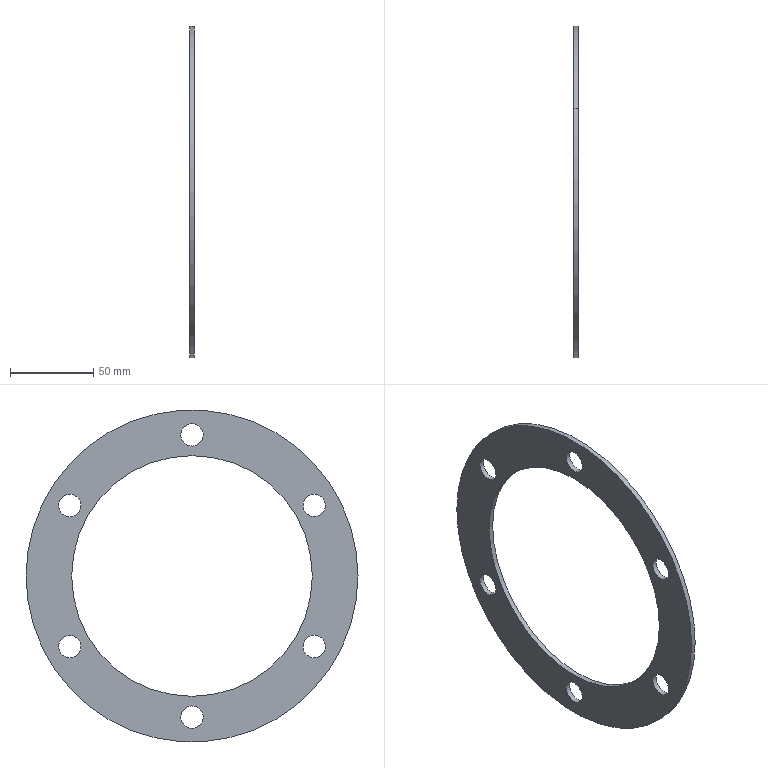Component | SolidWorks | JF21-80.1-33-1-SOLID1-1 | 1 solid | 18 faces | box 3 x 200 x 200 mm | volume 42132 mm3 | cylinder 16 | plane 2 | commonest cylinder face diameters 13.5 x12 145 x2 200 x2
STEP:
#1=COLOUR_RGB('',0.7922,0.8196,0.9333);
#2=FILL_AREA_STYLE_COLOUR('',#1);
#3=FILL_AREA_STYLE('',(#2));
#4=SURFACE_STYLE_FILL_AREA(#3);
#5=SURFACE_SIDE_STYLE('',(#4));
#6=SURFACE_STYLE_USAGE(.BOTH.,#5);
#7=PRESENTATION_STYLE_ASSIGNMENT((#6));
#8=CARTESIAN_POINT('',(17.244,-0.1329,18.038));
#9=VERTEX_POINT('',#8);
#10=CARTESIAN_POINT('',(17.244,0.1329,18.498));
#11=VERTEX_POINT('',#10);
#12=CARTESIAN_POINT('',(17.244,0.,18.268));
#13=DIRECTION('',(-1.,0.,0.));
#14=DIRECTION('',(0.,0.5,0.866));
#15=AXIS2_PLACEMENT_3D('',#12,#13,#14);
#16=CIRCLE('',#15,0.2657);
#17=EDGE_CURVE('',#9,#11,#16,.T.);
#18=ORIENTED_EDGE('',*,*,#17,.F.);
#19=CARTESIAN_POINT('',(17.126,-0.1329,18.038));
#20=VERTEX_POINT('',#19);
#21=CARTESIAN_POINT('',(17.126,-0.1329,18.038));
#22=DIRECTION('',(-1.,0.,0.));
#23=VECTOR('',#22,39.37);
#24=LINE('',#21,#23);
#25=EDGE_CURVE('',#9,#20,#24,.T.);
#26=ORIENTED_EDGE('',*,*,#25,.T.);
#27=CARTESIAN_POINT('',(17.126,0.1329,18.498));
#28=VERTEX_POINT('',#27);
#29=CARTESIAN_POINT('',(17.126,0.,18.268));
#30=DIRECTION('',(-1.,0.,0.));
#31=DIRECTION('',(0.,0.5,0.866));
#32=AXIS2_PLACEMENT_3D('',#29,#30,#31);
#33=CIRCLE('',#32,0.2657);
#34=EDGE_CURVE('',#20,#28,#33,.T.);
#35=ORIENTED_EDGE('',*,*,#34,.T.);
#36=CARTESIAN_POINT('',(17.126,0.1329,18.498));
#37=DIRECTION('',(-1.,0.,0.));
#38=VECTOR('',#37,39.37);
#39=LINE('',#36,#38);
#40=EDGE_CURVE('',#11,#28,#39,.T.);
#41=ORIENTED_EDGE('',*,*,#40,.F.);
#42=EDGE_LOOP('',(#18,#26,#35,#41));
#43=FACE_OUTER_BOUND('',#42,.T.);
#44=CARTESIAN_POINT('',(17.126,0.,18.268));
#45=DIRECTION('',(-1.,0.,0.));
#46=DIRECTION('',(0.,-0.5,-0.866));
#47=AXIS2_PLACEMENT_3D('',#44,#45,#46);
#48=CYLINDRICAL_SURFACE('',#47,0.2657);
#49=ADVANCED_FACE('',(#43),#48,.F.);
#50=CARTESIAN_POINT('',(17.244,-3.031,19.711));
#51=VERTEX_POINT('',#50);
#52=CARTESIAN_POINT('',(17.244,-2.765,20.171));
#53=VERTEX_POINT('',#52);
#54=CARTESIAN_POINT('',(17.244,-2.898,19.941));
#55=DIRECTION('',(-1.,0.,0.));
#56=DIRECTION('',(0.,0.5,0.866));
#57=AXIS2_PLACEMENT_3D('',#54,#55,#56);
#58=CIRCLE('',#57,0.2657);
#59=EDGE_CURVE('',#51,#53,#58,.T.);
#60=ORIENTED_EDGE('',*,*,#59,.F.);
#61=CARTESIAN_POINT('',(17.126,-3.031,19.711));
#62=VERTEX_POINT('',#61);
#63=CARTESIAN_POINT('',(17.126,-3.031,19.711));
#64=DIRECTION('',(-1.,0.,0.));
#65=VECTOR('',#64,39.37);
#66=LINE('',#63,#65);
#67=EDGE_CURVE('',#51,#62,#66,.T.);
#68=ORIENTED_EDGE('',*,*,#67,.T.);
#69=CARTESIAN_POINT('',(17.126,-2.765,20.171));
#70=VERTEX_POINT('',#69);
#71=CARTESIAN_POINT('',(17.126,-2.898,19.941));
#72=DIRECTION('',(-1.,0.,0.));
#73=DIRECTION('',(0.,0.5,0.866));
#74=AXIS2_PLACEMENT_3D('',#71,#72,#73);
#75=CIRCLE('',#74,0.2657);
#76=EDGE_CURVE('',#62,#70,#75,.T.);
#77=ORIENTED_EDGE('',*,*,#76,.T.);
#78=CARTESIAN_POINT('',(17.126,-2.765,20.171));
#79=DIRECTION('',(-1.,0.,0.));
#80=VECTOR('',#79,39.37);
#81=LINE('',#78,#80);
#82=EDGE_CURVE('',#53,#70,#81,.T.);
#83=ORIENTED_EDGE('',*,*,#82,.F.);
#84=EDGE_LOOP('',(#60,#68,#77,#83));
#85=FACE_OUTER_BOUND('',#84,.T.);
#86=CARTESIAN_POINT('',(17.126,-2.898,19.941));
#87=DIRECTION('',(-1.,0.,0.));
#88=DIRECTION('',(0.,-0.5,-0.866));
#89=AXIS2_PLACEMENT_3D('',#86,#87,#88);
#90=CYLINDRICAL_SURFACE('',#89,0.2657);
#91=ADVANCED_FACE('',(#85),#90,.F.);
#92=CARTESIAN_POINT('',(17.244,-3.031,23.057));
#93=VERTEX_POINT('',#92);
#94=CARTESIAN_POINT('',(17.244,-2.765,23.518));
#95=VERTEX_POINT('',#94);
#96=CARTESIAN_POINT('',(17.244,-2.898,23.287));
#97=DIRECTION('',(-1.,0.,0.));
#98=DIRECTION('',(0.,0.5,0.866));
#99=AXIS2_PLACEMENT_3D('',#96,#97,#98);
#100=CIRCLE('',#99,0.2657);
#101=EDGE_CURVE('',#93,#95,#100,.T.);
#102=ORIENTED_EDGE('',*,*,#101,.F.);
#103=CARTESIAN_POINT('',(17.126,-3.031,23.057));
#104=VERTEX_POINT('',#103);
#105=CARTESIAN_POINT('',(17.126,-3.031,23.057));
#106=DIRECTION('',(-1.,0.,0.));
#107=VECTOR('',#106,39.37);
#108=LINE('',#105,#107);
#109=EDGE_CURVE('',#93,#104,#108,.T.);
#110=ORIENTED_EDGE('',*,*,#109,.T.);
#111=CARTESIAN_POINT('',(17.126,-2.765,23.518));
#112=VERTEX_POINT('',#111);
#113=CARTESIAN_POINT('',(17.126,-2.898,23.287));
#114=DIRECTION('',(-1.,0.,0.));
#115=DIRECTION('',(0.,0.5,0.866));
#116=AXIS2_PLACEMENT_3D('',#113,#114,#115);
#117=CIRCLE('',#116,0.2657);
#118=EDGE_CURVE('',#104,#112,#117,.T.);
#119=ORIENTED_EDGE('',*,*,#118,.T.);
#120=CARTESIAN_POINT('',(17.126,-2.765,23.518));
#121=DIRECTION('',(-1.,0.,0.));
#122=VECTOR('',#121,39.37);
#123=LINE('',#120,#122);
#124=EDGE_CURVE('',#95,#112,#123,.T.);
#125=ORIENTED_EDGE('',*,*,#124,.F.);
#126=EDGE_LOOP('',(#102,#110,#119,#125));
#127=FACE_OUTER_BOUND('',#126,.T.);
#128=CARTESIAN_POINT('',(17.126,-2.898,23.287));
#129=DIRECTION('',(-1.,0.,0.));
#130=DIRECTION('',(0.,-0.5,-0.866));
#131=AXIS2_PLACEMENT_3D('',#128,#129,#130);
#132=CYLINDRICAL_SURFACE('',#131,0.2657);
#133=ADVANCED_FACE('',(#127),#132,.F.);
#134=CARTESIAN_POINT('',(17.244,-0.1329,24.73));
#135=VERTEX_POINT('',#134);
#136=CARTESIAN_POINT('',(17.244,0.1329,25.191));
#137=VERTEX_POINT('',#136);
#138=CARTESIAN_POINT('',(17.244,0.,24.961));
#139=DIRECTION('',(-1.,0.,0.));
#140=DIRECTION('',(0.,0.5,0.866));
#141=AXIS2_PLACEMENT_3D('',#138,#139,#140);
#142=CIRCLE('',#141,0.2657);
#143=EDGE_CURVE('',#135,#137,#142,.T.);
#144=ORIENTED_EDGE('',*,*,#143,.F.);
#145=CARTESIAN_POINT('',(17.126,-0.1329,24.73));
#146=VERTEX_POINT('',#145);
#147=CARTESIAN_POINT('',(17.126,-0.1329,24.73));
#148=DIRECTION('',(-1.,0.,0.));
#149=VECTOR('',#148,39.37);
#150=LINE('',#147,#149);
#151=EDGE_CURVE('',#135,#146,#150,.T.);
#152=ORIENTED_EDGE('',*,*,#151,.T.);
#153=CARTESIAN_POINT('',(17.126,0.1329,25.191));
#154=VERTEX_POINT('',#153);
#155=CARTESIAN_POINT('',(17.126,0.,24.961));
#156=DIRECTION('',(-1.,0.,0.));
#157=DIRECTION('',(0.,0.5,0.866));
#158=AXIS2_PLACEMENT_3D('',#155,#156,#157);
#159=CIRCLE('',#158,0.2657);
#160=EDGE_CURVE('',#146,#154,#159,.T.);
#161=ORIENTED_EDGE('',*,*,#160,.T.);
#162=CARTESIAN_POINT('',(17.126,0.1329,25.191));
#163=DIRECTION('',(-1.,0.,0.));
#164=VECTOR('',#163,39.37);
#165=LINE('',#162,#164);
#166=EDGE_CURVE('',#137,#154,#165,.T.);
#167=ORIENTED_EDGE('',*,*,#166,.F.);
#168=EDGE_LOOP('',(#144,#152,#161,#167));
#169=FACE_OUTER_BOUND('',#168,.T.);
#170=CARTESIAN_POINT('',(17.126,0.,24.961));
#171=DIRECTION('',(-1.,0.,0.));
#172=DIRECTION('',(0.,-0.5,-0.866));
#173=AXIS2_PLACEMENT_3D('',#170,#171,#172);
#174=CYLINDRICAL_SURFACE('',#173,0.2657);
#175=ADVANCED_FACE('',(#169),#174,.F.);
#176=CARTESIAN_POINT('',(17.244,2.765,23.057));
#177=VERTEX_POINT('',#176);
#178=CARTESIAN_POINT('',(17.244,3.031,23.518));
#179=VERTEX_POINT('',#178);
#180=CARTESIAN_POINT('',(17.244,2.898,23.287));
#181=DIRECTION('',(-1.,0.,0.));
#182=DIRECTION('',(0.,0.5,0.866));
#183=AXIS2_PLACEMENT_3D('',#180,#181,#182);
#184=CIRCLE('',#183,0.2657);
#185=EDGE_CURVE('',#177,#179,#184,.T.);
#186=ORIENTED_EDGE('',*,*,#185,.F.);
#187=CARTESIAN_POINT('',(17.126,2.765,23.057));
#188=VERTEX_POINT('',#187);
#189=CARTESIAN_POINT('',(17.126,2.765,23.057));
#190=DIRECTION('',(-1.,0.,0.));
#191=VECTOR('',#190,39.37);
#192=LINE('',#189,#191);
#193=EDGE_CURVE('',#177,#188,#192,.T.);
#194=ORIENTED_EDGE('',*,*,#193,.T.);
#195=CARTESIAN_POINT('',(17.126,3.031,23.518));
#196=VERTEX_POINT('',#195);
#197=CARTESIAN_POINT('',(17.126,2.898,23.287));
#198=DIRECTION('',(-1.,0.,0.));
#199=DIRECTION('',(0.,0.5,0.866));
#200=AXIS2_PLACEMENT_3D('',#197,#198,#199);
#201=CIRCLE('',#200,0.2657);
#202=EDGE_CURVE('',#188,#196,#201,.T.);
#203=ORIENTED_EDGE('',*,*,#202,.T.);
#204=CARTESIAN_POINT('',(17.126,3.031,23.518));
#205=DIRECTION('',(-1.,0.,0.));
#206=VECTOR('',#205,39.37);
#207=LINE('',#204,#206);
#208=EDGE_CURVE('',#179,#196,#207,.T.);
#209=ORIENTED_EDGE('',*,*,#208,.F.);
#210=EDGE_LOOP('',(#186,#194,#203,#209));
#211=FACE_OUTER_BOUND('',#210,.T.);
#212=CARTESIAN_POINT('',(17.126,2.898,23.287));
#213=DIRECTION('',(-1.,0.,0.));
#214=DIRECTION('',(0.,-0.5,-0.866));
#215=AXIS2_PLACEMENT_3D('',#212,#213,#214);
#216=CYLINDRICAL_SURFACE('',#215,0.2657);
#217=ADVANCED_FACE('',(#211),#216,.F.);
#218=CARTESIAN_POINT('',(17.244,2.765,19.711));
#219=VERTEX_POINT('',#218);
#220=CARTESIAN_POINT('',(17.244,3.031,20.171));
#221=VERTEX_POINT('',#220);
#222=CARTESIAN_POINT('',(17.244,2.898,19.941));
#223=DIRECTION('',(-1.,0.,0.));
#224=DIRECTION('',(0.,0.5,0.866));
#225=AXIS2_PLACEMENT_3D('',#222,#223,#224);
#226=CIRCLE('',#225,0.2657);
#227=EDGE_CURVE('',#219,#221,#226,.T.);
#228=ORIENTED_EDGE('',*,*,#227,.F.);
#229=CARTESIAN_POINT('',(17.126,2.765,19.711));
#230=VERTEX_POINT('',#229);
#231=CARTESIAN_POINT('',(17.126,2.765,19.711));
#232=DIRECTION('',(-1.,0.,0.));
#233=VECTOR('',#232,39.37);
#234=LINE('',#231,#233);
#235=EDGE_CURVE('',#219,#230,#234,.T.);
#236=ORIENTED_EDGE('',*,*,#235,.T.);
#237=CARTESIAN_POINT('',(17.126,3.031,20.171));
#238=VERTEX_POINT('',#237);
#239=CARTESIAN_POINT('',(17.126,2.898,19.941));
#240=DIRECTION('',(-1.,0.,0.));
#241=DIRECTION('',(0.,0.5,0.866));
#242=AXIS2_PLACEMENT_3D('',#239,#240,#241);
#243=CIRCLE('',#242,0.2657);
#244=EDGE_CURVE('',#230,#238,#243,.T.);
#245=ORIENTED_EDGE('',*,*,#244,.T.);
#246=CARTESIAN_POINT('',(17.126,3.031,20.171));
#247=DIRECTION('',(-1.,0.,0.));
#248=VECTOR('',#247,39.37);
#249=LINE('',#246,#248);
#250=EDGE_CURVE('',#221,#238,#249,.T.);
#251=ORIENTED_EDGE('',*,*,#250,.F.);
#252=EDGE_LOOP('',(#228,#236,#245,#251));
#253=FACE_OUTER_BOUND('',#252,.T.);
#254=CARTESIAN_POINT('',(17.126,2.898,19.941));
#255=DIRECTION('',(-1.,0.,0.));
#256=DIRECTION('',(0.,-0.5,-0.866));
#257=AXIS2_PLACEMENT_3D('',#254,#255,#256);
#258=CYLINDRICAL_SURFACE('',#257,0.2657);
#259=ADVANCED_FACE('',(#253),#258,.F.);
#260=CARTESIAN_POINT('',(17.126,-1.427,19.142));
#261=VERTEX_POINT('',#260);
#262=CARTESIAN_POINT('',(17.126,1.427,24.086));
#263=VERTEX_POINT('',#262);
#264=CARTESIAN_POINT('',(17.126,0.,21.614));
#265=DIRECTION('',(-1.,0.,0.));
#266=DIRECTION('',(0.,0.5,0.866));
#267=AXIS2_PLACEMENT_3D('',#264,#265,#266);
#268=CIRCLE('',#267,2.854);
#269=EDGE_CURVE('',#261,#263,#268,.T.);
#270=ORIENTED_EDGE('',*,*,#269,.T.);
#271=CARTESIAN_POINT('',(17.244,1.427,24.086));
#272=VERTEX_POINT('',#271);
#273=CARTESIAN_POINT('',(17.126,1.427,24.086));
#274=DIRECTION('',(-1.,0.,0.));
#275=VECTOR('',#274,39.37);
#276=LINE('',#273,#275);
#277=EDGE_CURVE('',#272,#263,#276,.T.);
#278=ORIENTED_EDGE('',*,*,#277,.F.);
#279=CARTESIAN_POINT('',(17.244,-1.427,19.142));
#280=VERTEX_POINT('',#279);
#281=CARTESIAN_POINT('',(17.244,0.,21.614));
#282=DIRECTION('',(-1.,0.,0.));
#283=DIRECTION('',(0.,0.5,0.866));
#284=AXIS2_PLACEMENT_3D('',#281,#282,#283);
#285=CIRCLE('',#284,2.854);
#286=EDGE_CURVE('',#280,#272,#285,.T.);
#287=ORIENTED_EDGE('',*,*,#286,.F.);
#288=CARTESIAN_POINT('',(17.126,-1.427,19.142));
#289=DIRECTION('',(-1.,0.,0.));
#290=VECTOR('',#289,39.37);
#291=LINE('',#288,#290);
#292=EDGE_CURVE('',#280,#261,#291,.T.);
#293=ORIENTED_EDGE('',*,*,#292,.T.);
#294=EDGE_LOOP('',(#270,#278,#287,#293));
#295=FACE_OUTER_BOUND('',#294,.T.);
#296=CARTESIAN_POINT('',(17.126,0.,21.614));
#297=DIRECTION('',(1.,0.,0.));
#298=DIRECTION('',(0.,0.5,0.866));
#299=AXIS2_PLACEMENT_3D('',#296,#297,#298);
#300=CYLINDRICAL_SURFACE('',#299,2.854);
#301=ADVANCED_FACE('',(#295),#300,.F.);
#302=CARTESIAN_POINT('',(17.126,1.969,25.024));
#303=VERTEX_POINT('',#302);
#304=CARTESIAN_POINT('',(17.126,-1.969,18.205));
#305=VERTEX_POINT('',#304);
#306=CARTESIAN_POINT('',(17.126,0.,21.614));
#307=DIRECTION('',(-1.,0.,0.));
#308=DIRECTION('',(0.,0.5,0.866));
#309=AXIS2_PLACEMENT_3D('',#306,#307,#308);
#310=CIRCLE('',#309,3.937);
#311=EDGE_CURVE('',#303,#305,#310,.T.);
#312=ORIENTED_EDGE('',*,*,#311,.F.);
#313=CARTESIAN_POINT('',(17.244,1.969,25.024));
#314=VERTEX_POINT('',#313);
#315=CARTESIAN_POINT('',(17.126,1.969,25.024));
#316=DIRECTION('',(-1.,0.,0.));
#317=VECTOR('',#316,39.37);
#318=LINE('',#315,#317);
#319=EDGE_CURVE('',#314,#303,#318,.T.);
#320=ORIENTED_EDGE('',*,*,#319,.F.);
#321=CARTESIAN_POINT('',(17.244,-1.969,18.205));
#322=VERTEX_POINT('',#321);
#323=CARTESIAN_POINT('',(17.244,0.,21.614));
#324=DIRECTION('',(-1.,0.,0.));
#325=DIRECTION('',(0.,0.5,0.866));
#326=AXIS2_PLACEMENT_3D('',#323,#324,#325);
#327=CIRCLE('',#326,3.937);
#328=EDGE_CURVE('',#314,#322,#327,.T.);
#329=ORIENTED_EDGE('',*,*,#328,.T.);
#330=CARTESIAN_POINT('',(17.126,-1.969,18.205));
#331=DIRECTION('',(-1.,0.,0.));
#332=VECTOR('',#331,39.37);
#333=LINE('',#330,#332);
#334=EDGE_CURVE('',#322,#305,#333,.T.);
#335=ORIENTED_EDGE('',*,*,#334,.T.);
#336=EDGE_LOOP('',(#312,#320,#329,#335));
#337=FACE_OUTER_BOUND('',#336,.T.);
#338=CARTESIAN_POINT('',(17.126,0.,21.614));
#339=DIRECTION('',(1.,0.,0.));
#340=DIRECTION('',(0.,0.5,0.866));
#341=AXIS2_PLACEMENT_3D('',#338,#339,#340);
#342=CYLINDRICAL_SURFACE('',#341,3.937);
#343=ADVANCED_FACE('',(#337),#342,.T.);
#344=CARTESIAN_POINT('',(17.126,0.,18.268));
#345=DIRECTION('',(-1.,0.,0.));
#346=DIRECTION('',(0.,0.5,0.866));
#347=AXIS2_PLACEMENT_3D('',#344,#345,#346);
#348=CIRCLE('',#347,0.2657);
#349=EDGE_CURVE('',#28,#20,#348,.T.);
#350=ORIENTED_EDGE('',*,*,#349,.F.);
#351=ORIENTED_EDGE('',*,*,#34,.F.);
#352=EDGE_LOOP('',(#350,#351));
#353=FACE_BOUND('',#352,.T.);
#354=CARTESIAN_POINT('',(17.126,-2.898,19.941));
#355=DIRECTION('',(-1.,0.,0.));
#356=DIRECTION('',(0.,0.5,0.866));
#357=AXIS2_PLACEMENT_3D('',#354,#355,#356);
#358=CIRCLE('',#357,0.2657);
#359=EDGE_CURVE('',#70,#62,#358,.T.);
#360=ORIENTED_EDGE('',*,*,#359,.F.);
#361=ORIENTED_EDGE('',*,*,#76,.F.);
#362=EDGE_LOOP('',(#360,#361));
#363=FACE_BOUND('',#362,.T.);
#364=CARTESIAN_POINT('',(17.126,-2.898,23.287));
#365=DIRECTION('',(-1.,0.,0.));
#366=DIRECTION('',(0.,0.5,0.866));
#367=AXIS2_PLACEMENT_3D('',#364,#365,#366);
#368=CIRCLE('',#367,0.2657);
#369=EDGE_CURVE('',#112,#104,#368,.T.);
#370=ORIENTED_EDGE('',*,*,#369,.F.);
#371=ORIENTED_EDGE('',*,*,#118,.F.);
#372=EDGE_LOOP('',(#370,#371));
#373=FACE_BOUND('',#372,.T.);
#374=CARTESIAN_POINT('',(17.126,0.,24.961));
#375=DIRECTION('',(-1.,0.,0.));
#376=DIRECTION('',(0.,0.5,0.866));
#377=AXIS2_PLACEMENT_3D('',#374,#375,#376);
#378=CIRCLE('',#377,0.2657);
#379=EDGE_CURVE('',#154,#146,#378,.T.);
#380=ORIENTED_EDGE('',*,*,#379,.F.);
#381=ORIENTED_EDGE('',*,*,#160,.F.);
#382=EDGE_LOOP('',(#380,#381));
#383=FACE_BOUND('',#382,.T.);
#384=CARTESIAN_POINT('',(17.126,2.898,23.287));
#385=DIRECTION('',(-1.,0.,0.));
#386=DIRECTION('',(0.,0.5,0.866));
#387=AXIS2_PLACEMENT_3D('',#384,#385,#386);
#388=CIRCLE('',#387,0.2657);
#389=EDGE_CURVE('',#196,#188,#388,.T.);
#390=ORIENTED_EDGE('',*,*,#389,.F.);
#391=ORIENTED_EDGE('',*,*,#202,.F.);
#392=EDGE_LOOP('',(#390,#391));
#393=FACE_BOUND('',#392,.T.);
#394=CARTESIAN_POINT('',(17.126,2.898,19.941));
#395=DIRECTION('',(-1.,0.,0.));
#396=DIRECTION('',(0.,0.5,0.866));
#397=AXIS2_PLACEMENT_3D('',#394,#395,#396);
#398=CIRCLE('',#397,0.2657);
#399=EDGE_CURVE('',#238,#230,#398,.T.);
#400=ORIENTED_EDGE('',*,*,#399,.F.);
#401=ORIENTED_EDGE('',*,*,#244,.F.);
#402=EDGE_LOOP('',(#400,#401));
#403=FACE_BOUND('',#402,.T.);
#404=CARTESIAN_POINT('',(17.126,0.,21.614));
#405=DIRECTION('',(-1.,0.,0.));
#406=DIRECTION('',(0.,0.5,0.866));
#407=AXIS2_PLACEMENT_3D('',#404,#405,#406);
#408=CIRCLE('',#407,3.937);
#409=EDGE_CURVE('',#305,#303,#408,.T.);
#410=ORIENTED_EDGE('',*,*,#409,.T.);
#411=ORIENTED_EDGE('',*,*,#311,.T.);
#412=EDGE_LOOP('',(#410,#411));
#413=FACE_OUTER_BOUND('',#412,.T.);
#414=ORIENTED_EDGE('',*,*,#269,.F.);
#415=CARTESIAN_POINT('',(17.126,0.,21.614));
#416=DIRECTION('',(-1.,0.,0.));
#417=DIRECTION('',(0.,0.5,0.866));
#418=AXIS2_PLACEMENT_3D('',#415,#416,#417);
#419=CIRCLE('',#418,2.854);
#420=EDGE_CURVE('',#263,#261,#419,.T.);
#421=ORIENTED_EDGE('',*,*,#420,.F.);
#422=EDGE_LOOP('',(#414,#421));
#423=FACE_BOUND('',#422,.T.);
#424=CARTESIAN_POINT('',(17.126,0.,21.614));
#425=DIRECTION('',(-1.,0.,0.));
#426=DIRECTION('',(0.,-0.5,-0.866));
#427=AXIS2_PLACEMENT_3D('',#424,#425,#426);
#428=PLANE('',#427);
#429=ADVANCED_FACE('',(#353,#363,#373,#383,#393,#403,#413,#423),#428,.T.);
#430=CARTESIAN_POINT('',(17.244,0.,18.268));
#431=DIRECTION('',(-1.,0.,0.));
#432=DIRECTION('',(0.,0.5,0.866));
#433=AXIS2_PLACEMENT_3D('',#430,#431,#432);
#434=CIRCLE('',#433,0.2657);
#435=EDGE_CURVE('',#11,#9,#434,.T.);
#436=ORIENTED_EDGE('',*,*,#435,.T.);
#437=ORIENTED_EDGE('',*,*,#17,.T.);
#438=EDGE_LOOP('',(#436,#437));
#439=FACE_BOUND('',#438,.T.);
#440=CARTESIAN_POINT('',(17.244,-2.898,19.941));
#441=DIRECTION('',(-1.,0.,0.));
#442=DIRECTION('',(0.,0.5,0.866));
#443=AXIS2_PLACEMENT_3D('',#440,#441,#442);
#444=CIRCLE('',#443,0.2657);
#445=EDGE_CURVE('',#53,#51,#444,.T.);
#446=ORIENTED_EDGE('',*,*,#445,.T.);
#447=ORIENTED_EDGE('',*,*,#59,.T.);
#448=EDGE_LOOP('',(#446,#447));
#449=FACE_BOUND('',#448,.T.);
#450=CARTESIAN_POINT('',(17.244,-2.898,23.287));
#451=DIRECTION('',(-1.,0.,0.));
#452=DIRECTION('',(0.,0.5,0.866));
#453=AXIS2_PLACEMENT_3D('',#450,#451,#452);
#454=CIRCLE('',#453,0.2657);
#455=EDGE_CURVE('',#95,#93,#454,.T.);
#456=ORIENTED_EDGE('',*,*,#455,.T.);
#457=ORIENTED_EDGE('',*,*,#101,.T.);
#458=EDGE_LOOP('',(#456,#457));
#459=FACE_BOUND('',#458,.T.);
#460=CARTESIAN_POINT('',(17.244,0.,24.961));
#461=DIRECTION('',(-1.,0.,0.));
#462=DIRECTION('',(0.,0.5,0.866));
#463=AXIS2_PLACEMENT_3D('',#460,#461,#462);
#464=CIRCLE('',#463,0.2657);
#465=EDGE_CURVE('',#137,#135,#464,.T.);
#466=ORIENTED_EDGE('',*,*,#465,.T.);
#467=ORIENTED_EDGE('',*,*,#143,.T.);
#468=EDGE_LOOP('',(#466,#467));
#469=FACE_BOUND('',#468,.T.);
#470=CARTESIAN_POINT('',(17.244,2.898,23.287));
#471=DIRECTION('',(-1.,0.,0.));
#472=DIRECTION('',(0.,0.5,0.866));
#473=AXIS2_PLACEMENT_3D('',#470,#471,#472);
#474=CIRCLE('',#473,0.2657);
#475=EDGE_CURVE('',#179,#177,#474,.T.);
#476=ORIENTED_EDGE('',*,*,#475,.T.);
#477=ORIENTED_EDGE('',*,*,#185,.T.);
#478=EDGE_LOOP('',(#476,#477));
#479=FACE_BOUND('',#478,.T.);
#480=CARTESIAN_POINT('',(17.244,2.898,19.941));
#481=DIRECTION('',(-1.,0.,0.));
#482=DIRECTION('',(0.,0.5,0.866));
#483=AXIS2_PLACEMENT_3D('',#480,#481,#482);
#484=CIRCLE('',#483,0.2657);
#485=EDGE_CURVE('',#221,#219,#484,.T.);
#486=ORIENTED_EDGE('',*,*,#485,.T.);
#487=ORIENTED_EDGE('',*,*,#227,.T.);
#488=EDGE_LOOP('',(#486,#487));
#489=FACE_BOUND('',#488,.T.);
#490=CARTESIAN_POINT('',(17.244,0.,21.614));
#491=DIRECTION('',(-1.,0.,0.));
#492=DIRECTION('',(0.,0.5,0.866));
#493=AXIS2_PLACEMENT_3D('',#490,#491,#492);
#494=CIRCLE('',#493,3.937);
#495=EDGE_CURVE('',#322,#314,#494,.T.);
#496=ORIENTED_EDGE('',*,*,#495,.F.);
#497=ORIENTED_EDGE('',*,*,#328,.F.);
#498=EDGE_LOOP('',(#496,#497));
#499=FACE_OUTER_BOUND('',#498,.T.);
#500=ORIENTED_EDGE('',*,*,#286,.T.);
#501=CARTESIAN_POINT('',(17.244,0.,21.614));
#502=DIRECTION('',(-1.,0.,0.));
#503=DIRECTION('',(0.,0.5,0.866));
#504=AXIS2_PLACEMENT_3D('',#501,#502,#503);
#505=CIRCLE('',#504,2.854);
#506=EDGE_CURVE('',#272,#280,#505,.T.);
#507=ORIENTED_EDGE('',*,*,#506,.T.);
#508=EDGE_LOOP('',(#500,#507));
#509=FACE_BOUND('',#508,.T.);
#510=CARTESIAN_POINT('',(17.244,0.,21.614));
#511=DIRECTION('',(-1.,0.,0.));
#512=DIRECTION('',(0.,-0.5,-0.866));
#513=AXIS2_PLACEMENT_3D('',#510,#511,#512);
#514=PLANE('',#513);
#515=ADVANCED_FACE('',(#439,#449,#459,#469,#479,#489,#499,#509),#514,.F.);
#516=ORIENTED_EDGE('',*,*,#319,.T.);
#517=ORIENTED_EDGE('',*,*,#409,.F.);
#518=ORIENTED_EDGE('',*,*,#334,.F.);
#519=ORIENTED_EDGE('',*,*,#495,.T.);
#520=EDGE_LOOP('',(#516,#517,#518,#519));
#521=FACE_OUTER_BOUND('',#520,.T.);
#522=CARTESIAN_POINT('',(17.126,0.,21.614));
#523=DIRECTION('',(1.,0.,0.));
#524=DIRECTION('',(0.,0.5,0.866));
#525=AXIS2_PLACEMENT_3D('',#522,#523,#524);
#526=CYLINDRICAL_SURFACE('',#525,3.937);
#527=ADVANCED_FACE('',(#521),#526,.T.);
#528=ORIENTED_EDGE('',*,*,#277,.T.);
#529=ORIENTED_EDGE('',*,*,#420,.T.);
#530=ORIENTED_EDGE('',*,*,#292,.F.);
#531=ORIENTED_EDGE('',*,*,#506,.F.);
#532=EDGE_LOOP('',(#528,#529,#530,#531));
#533=FACE_OUTER_BOUND('',#532,.T.);
#534=CARTESIAN_POINT('',(17.126,0.,21.614));
#535=DIRECTION('',(1.,0.,0.));
#536=DIRECTION('',(0.,0.5,0.866));
#537=AXIS2_PLACEMENT_3D('',#534,#535,#536);
#538=CYLINDRICAL_SURFACE('',#537,2.854);
#539=ADVANCED_FACE('',(#533),#538,.F.);
#540=ORIENTED_EDGE('',*,*,#235,.F.);
#541=ORIENTED_EDGE('',*,*,#485,.F.);
#542=ORIENTED_EDGE('',*,*,#250,.T.);
#543=ORIENTED_EDGE('',*,*,#399,.T.);
#544=EDGE_LOOP('',(#540,#541,#542,#543));
#545=FACE_OUTER_BOUND('',#544,.T.);
#546=CARTESIAN_POINT('',(17.126,2.898,19.941));
#547=DIRECTION('',(-1.,0.,0.));
#548=DIRECTION('',(0.,-0.5,-0.866));
#549=AXIS2_PLACEMENT_3D('',#546,#547,#548);
#550=CYLINDRICAL_SURFACE('',#549,0.2657);
#551=ADVANCED_FACE('',(#545),#550,.F.);
#552=ORIENTED_EDGE('',*,*,#193,.F.);
#553=ORIENTED_EDGE('',*,*,#475,.F.);
#554=ORIENTED_EDGE('',*,*,#208,.T.);
#555=ORIENTED_EDGE('',*,*,#389,.T.);
#556=EDGE_LOOP('',(#552,#553,#554,#555));
#557=FACE_OUTER_BOUND('',#556,.T.);
#558=CARTESIAN_POINT('',(17.126,2.898,23.287));
#559=DIRECTION('',(-1.,0.,0.));
#560=DIRECTION('',(0.,-0.5,-0.866));
#561=AXIS2_PLACEMENT_3D('',#558,#559,#560);
#562=CYLINDRICAL_SURFACE('',#561,0.2657);
#563=ADVANCED_FACE('',(#557),#562,.F.);
#564=ORIENTED_EDGE('',*,*,#151,.F.);
#565=ORIENTED_EDGE('',*,*,#465,.F.);
#566=ORIENTED_EDGE('',*,*,#166,.T.);
#567=ORIENTED_EDGE('',*,*,#379,.T.);
#568=EDGE_LOOP('',(#564,#565,#566,#567));
#569=FACE_OUTER_BOUND('',#568,.T.);
#570=CARTESIAN_POINT('',(17.126,0.,24.961));
#571=DIRECTION('',(-1.,0.,0.));
#572=DIRECTION('',(0.,-0.5,-0.866));
#573=AXIS2_PLACEMENT_3D('',#570,#571,#572);
#574=CYLINDRICAL_SURFACE('',#573,0.2657);
#575=ADVANCED_FACE('',(#569),#574,.F.);
#576=ORIENTED_EDGE('',*,*,#109,.F.);
#577=ORIENTED_EDGE('',*,*,#455,.F.);
#578=ORIENTED_EDGE('',*,*,#124,.T.);
#579=ORIENTED_EDGE('',*,*,#369,.T.);
#580=EDGE_LOOP('',(#576,#577,#578,#579));
#581=FACE_OUTER_BOUND('',#580,.T.);
#582=CARTESIAN_POINT('',(17.126,-2.898,23.287));
#583=DIRECTION('',(-1.,0.,0.));
#584=DIRECTION('',(0.,-0.5,-0.866));
#585=AXIS2_PLACEMENT_3D('',#582,#583,#584);
#586=CYLINDRICAL_SURFACE('',#585,0.2657);
#587=ADVANCED_FACE('',(#581),#586,.F.);
#588=ORIENTED_EDGE('',*,*,#67,.F.);
#589=ORIENTED_EDGE('',*,*,#445,.F.);
#590=ORIENTED_EDGE('',*,*,#82,.T.);
#591=ORIENTED_EDGE('',*,*,#359,.T.);
#592=EDGE_LOOP('',(#588,#589,#590,#591));
#593=FACE_OUTER_BOUND('',#592,.T.);
#594=CARTESIAN_POINT('',(17.126,-2.898,19.941));
#595=DIRECTION('',(-1.,0.,0.));
#596=DIRECTION('',(0.,-0.5,-0.866));
#597=AXIS2_PLACEMENT_3D('',#594,#595,#596);
#598=CYLINDRICAL_SURFACE('',#597,0.2657);
#599=ADVANCED_FACE('',(#593),#598,.F.);
#600=ORIENTED_EDGE('',*,*,#25,.F.);
#601=ORIENTED_EDGE('',*,*,#435,.F.);
#602=ORIENTED_EDGE('',*,*,#40,.T.);
#603=ORIENTED_EDGE('',*,*,#349,.T.);
#604=EDGE_LOOP('',(#600,#601,#602,#603));
#605=FACE_OUTER_BOUND('',#604,.T.);
#606=CARTESIAN_POINT('',(17.126,0.,18.268));
#607=DIRECTION('',(-1.,0.,0.));
#608=DIRECTION('',(0.,-0.5,-0.866));
#609=AXIS2_PLACEMENT_3D('',#606,#607,#608);
#610=CYLINDRICAL_SURFACE('',#609,0.2657);
#611=ADVANCED_FACE('',(#605),#610,.F.);
#612=CLOSED_SHELL('',(#49,#91,#133,#175,#217,#259,#301,#343,#429,#515,#527,#539,#551,#563,#575,#587,#599,#611));
#613=MANIFOLD_SOLID_BREP('',#612);
#614=STYLED_ITEM('',(#7),#613);
#615=PRESENTATION_LAYER_ASSIGNMENT('','',(#614));
#616=CARTESIAN_POINT('',(0.,0.,0.));
#617=DIRECTION('',(0.,0.,1.));
#618=DIRECTION('',(1.,0.,0.));
#619=AXIS2_PLACEMENT_3D('',#616,#617,#618);
#620=(LENGTH_UNIT()NAMED_UNIT(*)SI_UNIT($,.METRE.));
#621=LENGTH_MEASURE_WITH_UNIT(LENGTH_MEASURE(0.0254),#620);
#622=DIMENSIONAL_EXPONENTS(1.,0.,0.,0.,0.,0.,0.);
#623=(CONVERSION_BASED_UNIT('',#621)LENGTH_UNIT()NAMED_UNIT(#622));
#624=UNCERTAINTY_MEASURE_WITH_UNIT(LENGTH_MEASURE(0.00001),#623,'','');
#625=(NAMED_UNIT(*)PLANE_ANGLE_UNIT()SI_UNIT($,.RADIAN.));
#626=(NAMED_UNIT(*)SI_UNIT($,.STERADIAN.)SOLID_ANGLE_UNIT());
#627=(GEOMETRIC_REPRESENTATION_CONTEXT(3)GLOBAL_UNCERTAINTY_ASSIGNED_CONTEXT((#624))GLOBAL_UNIT_ASSIGNED_CONTEXT((#623,#625,#626))REPRESENTATION_CONTEXT('',''));
#628=ADVANCED_BREP_SHAPE_REPRESENTATION('',(#613,#619),#627);
#629=(LENGTH_UNIT()NAMED_UNIT(*)SI_UNIT($,.METRE.));
#630=LENGTH_MEASURE_WITH_UNIT(LENGTH_MEASURE(0.0254),#629);
#631=DIMENSIONAL_EXPONENTS(1.,0.,0.,0.,0.,0.,0.);
#632=(CONVERSION_BASED_UNIT('',#630)LENGTH_UNIT()NAMED_UNIT(#631));
#633=UNCERTAINTY_MEASURE_WITH_UNIT(LENGTH_MEASURE(0.00001),#632,'','');
#634=(NAMED_UNIT(*)PLANE_ANGLE_UNIT()SI_UNIT($,.RADIAN.));
#635=(NAMED_UNIT(*)SI_UNIT($,.STERADIAN.)SOLID_ANGLE_UNIT());
#636=(GEOMETRIC_REPRESENTATION_CONTEXT(3)GLOBAL_UNCERTAINTY_ASSIGNED_CONTEXT((#633))GLOBAL_UNIT_ASSIGNED_CONTEXT((#632,#634,#635))REPRESENTATION_CONTEXT('',''));
#637=MECHANICAL_DESIGN_GEOMETRIC_PRESENTATION_REPRESENTATION('',(#614),#636);